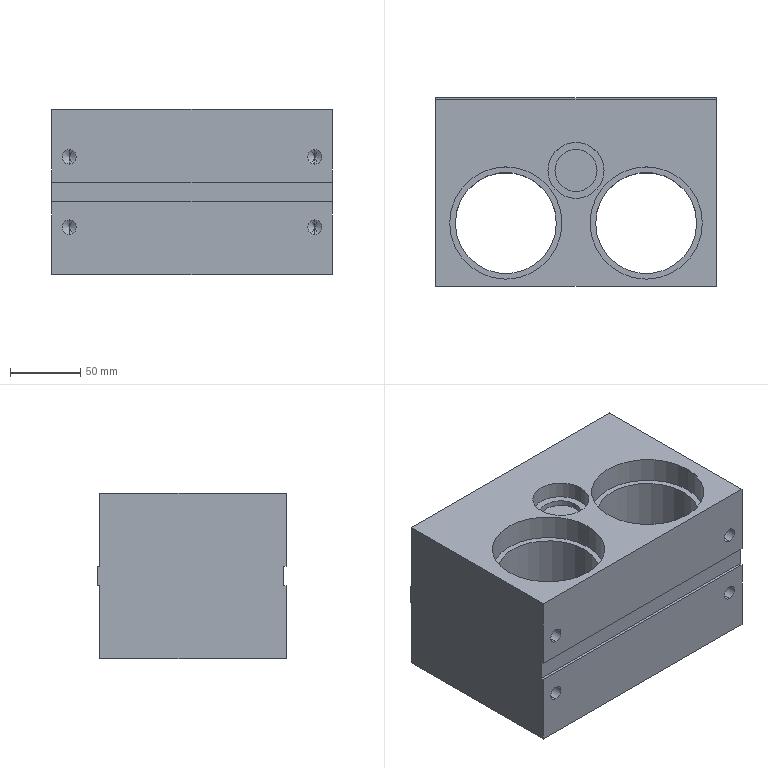Component | SolidWorks | NewTypeCurveBenderReinforcementSeatUpperWheelBox4-DoubleWheel-1 | 1 solid | 68 faces | box 200 x 134.5 x 118 mm | volume 2070066 mm3 | cylinder 32 | plane 20 | cone 16 | commonest cylinder face diameters 10.2 x16 80 x8 72 x4 30 x2 40 x2
build123d program:
from build123d import *

# Parameters (mm, degrees)
SKETCH1_W              = 200
SKETCH1_H              = 118
BOSS_EXTRUDE1_DEPTH    = 133
SKETCH2_R              = 36
CUT_EXTRUDE1_DEPTH     = 138
SKETCH3_R              = 40
CUT_EXTRUDE2_DEPTH     = 18
CUT_EXTRUDE3_START     = -18
SKETCH4_R              = 40
CUT_EXTRUDE3_DEPTH     = 18
SKETCH5_R              = 20
CUT_EXTRUDE4_DEPTH     = 12
SKETCH6_R              = 15
CUT_EXTRUDE5_DEPTH     = 4
M12_TAPPED_HOLE1_D     = 10.2
M12_TAPPED_HOLE1_DEPTH = 29.25
M12_TAPPED_HOLE1_TIP   = 3.064
M12_TAPPED_HOLE2_D     = 10.2
M12_TAPPED_HOLE2_DEPTH = 29.25
M12_TAPPED_HOLE2_TIP   = 3.064
SKETCH11_W             = 14
SKETCH11_H             = 1.5
BOSS_EXTRUDE2_DEPTH    = 200
SKETCH12_W             = 14
SKETCH12_H             = 4
CUT_EXTRUDE6_DEPTH     = 248.326


with BuildPart() as part:
    # Sketch1 → Boss-Extrude1 (new body)
    with BuildSketch(Plane(origin=(0, 0, 0), x_dir=(1, 0, 0), z_dir=(0, 1, 0))):
        Rectangle(SKETCH1_W, SKETCH1_H)
    extrude(amount=BOSS_EXTRUDE1_DEPTH)

    # Sketch2 → Cut-Extrude1 (cut)
    with BuildSketch(Plane.XY.offset(59)):
        with Locations((-50, 88)):
            Circle(SKETCH2_R)
        with Locations((50, 88)):
            Circle(SKETCH2_R)
    extrude(amount=-CUT_EXTRUDE1_DEPTH, mode=Mode.SUBTRACT)

    # Sketch3 → Cut-Extrude2 (cut)
    with BuildSketch(Plane.XY.offset(59)):
        with Locations((-50, 88)):
            Circle(SKETCH3_R)
        with Locations((50, 88)):
            Circle(SKETCH3_R)
    extrude(amount=-CUT_EXTRUDE2_DEPTH, mode=Mode.SUBTRACT)

    # Sketch4 → Cut-Extrude3 (cut)
    with BuildSketch(Plane(origin=(0, 0, -59), x_dir=(-1, 0, 0), z_dir=(0, 0, -1)).offset(CUT_EXTRUDE3_START)):
        with Locations(Location((-50, 88, 0), (0, 0, 180))):
            Circle(SKETCH4_R)
        with Locations(Location((50, 88, 0), (0, 0, 180))):
            Circle(SKETCH4_R)
    extrude(amount=CUT_EXTRUDE3_DEPTH, mode=Mode.SUBTRACT)

    # Sketch5 → Cut-Extrude4 (cut)
    with BuildSketch(Plane.XY.offset(59)):
        with Locations((0, 50.5)):
            Circle(SKETCH5_R)
    extrude(amount=-CUT_EXTRUDE4_DEPTH, mode=Mode.SUBTRACT)

    # Sketch6 → Cut-Extrude5 (cut)
    with BuildSketch(Plane.XY.offset(47)):
        with Locations((0, 50.5)):
            Circle(SKETCH6_R)
    extrude(amount=-CUT_EXTRUDE5_DEPTH, mode=Mode.SUBTRACT)

    # M12 Tapped Hole1
    with Locations(Plane(origin=(0, 0, 0), x_dir=(-1, 0, 0), z_dir=(0, -1, 0))):
        with Locations((-90, 45), (-90, -45), (90, 45), (90, -45)):
            Hole(M12_TAPPED_HOLE1_D / 2, depth=M12_TAPPED_HOLE1_DEPTH)
            with Locations((0, 0, -(M12_TAPPED_HOLE1_DEPTH + M12_TAPPED_HOLE1_TIP / 2))):  # 118° drill point
                Cone(0, M12_TAPPED_HOLE1_D / 2, M12_TAPPED_HOLE1_TIP, mode=Mode.SUBTRACT)

    # M12 Tapped Hole2
    with Locations(Plane(origin=(0, 133, 0), x_dir=(1, 0, 0), z_dir=(0, 1, 0))):
        with Locations((-87.5, 25), (-87.5, -25), (87.5, 25), (87.5, -25)):
            Hole(M12_TAPPED_HOLE2_D / 2, depth=M12_TAPPED_HOLE2_DEPTH)
            with Locations((0, 0, -(M12_TAPPED_HOLE2_DEPTH + M12_TAPPED_HOLE2_TIP / 2))):  # 118° drill point
                Cone(0, M12_TAPPED_HOLE2_D / 2, M12_TAPPED_HOLE2_TIP, mode=Mode.SUBTRACT)

    # Sketch11 → Boss-Extrude2 (add)
    with BuildSketch(Plane.ZY.offset(100)):
        with Locations((0, -0.75)):
            Rectangle(SKETCH11_W, SKETCH11_H)
    extrude(amount=-BOSS_EXTRUDE2_DEPTH)

    # Sketch12 → Cut-Extrude6 (cut, through all)
    with BuildSketch(Plane.ZY.offset(100)):
        with Locations((0, 133)):
            Rectangle(SKETCH12_W, SKETCH12_H)
    extrude(amount=-CUT_EXTRUDE6_DEPTH, mode=Mode.SUBTRACT)


solid = part.part

# Placed as in the assembly
solid = solid.moved(Location((0, 0, 0), (0, 0, 180)))